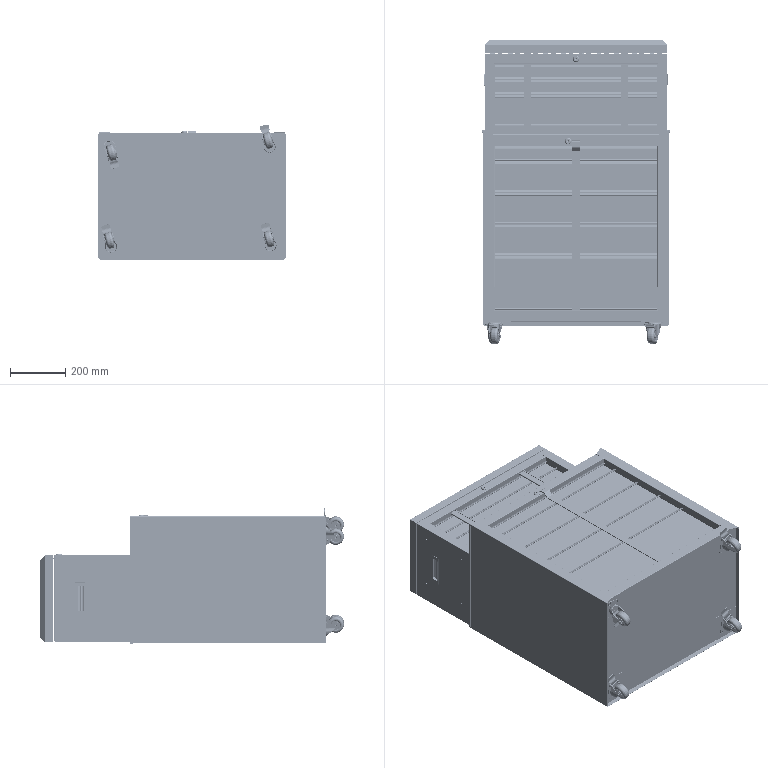Assembly | SolidWorks | mm | 91 component files | 95 solids | 8380 faces | box 675.6 x 1097.13 x 487.94 mm | volume 6787834 mm3 | plane 4464 | cylinder 3108 | spline 614 | torus 142 | cone 52 | commonest cylinder face diameters 4 x508 1 x387 2 x248 8 x224 3 x199 4.7 x186 5 x164 2.4 x130
Bill of materials:
Chapa Guantera Duesco | 2 | Plain Carbon Steel | Short cylindrical body with a wider flanged head with a chamfered edge. The shank has helical thread-like grooves interrupted by two flats on opposite sides. The end face has a slotted keyway-style recess, and a small rectangular tab sticks out of the opposite end.
Corredera A 400 | 10 | Plain Carbon Steel | Long, narrow formed channel (C-profile) with rounded bends and short return lips. The web has a row of pierced features: rectangular hook-like cut-outs, each with small round holes and slots around it, set in two groups near each end. There are notches at the ends.
Lengueta Chapa Guantera Duesco B | 1 | Plain Carbon Steel | Flat obround (stadium-shaped) plate with an eight-point star-shaped through cut-out near one end. A small cylindrical pin sits at the centre of the cut-out and sticks out a little below the plate.
Corredera C 400 | 10 | Plain Carbon Steel | Long, slender formed channel with rounded bends and short return flanges. It has three evenly spaced groups of small perforations along the web and a notch at one end.
PM-CAJ-P51 | 3 | Plain Carbon Steel | Long, narrow formed sheet profile. A flat base runs into an angled step and an upright leg at one edge. At the other edge it bends up into a side wall that ends in a folded-back (hemmed) angled lip. There are no visible holes.
PM-CAJ-P56 | 1 | Plain Carbon Steel | Rectangular sheet panel with a narrow perpendicular flange along one short edge. The flange has three small round holes in a line. There is also a small folded return along the top edge at one corner.
PM-CAJ-P54 | 4 | Plain Carbon Steel | Long formed sheet profile with a wide flat base. One edge has an angled step and an upright leg. The other edge has a vertical wall ending in a hemmed angled lip. There are no visible holes.
PM-CAJ-P57 | 3 | Plain Carbon Steel | Rectangular sheet panel with right-angle flanges along both short edges, forming a shallow U or tray shape seen from above. Each flange has three small round holes in a line.
PM-CAJ-P58 | 1 | Plain Carbon Steel | Rectangular sheet panel with deep right-angle flanges along both short edges, forming a U-shaped shell. Each flange has three small round holes in a line.
PM-CAJ-P59 | 1 | Plain Carbon Steel | Wide, long formed sheet profile. A large flat base has an angled step and an upright leg at one edge, and a vertical wall with a hemmed angled lip at the other edge. There are no visible holes.
PM-CAJ-P33 | 1 | Plain Carbon Steel | Rectangular sheet panel. Shallow flanges are folded along the bottom edge and both side edges, and the top edge has a folded channel-like return (a U-shaped hook). There are no visible holes.
PM-CAJ-P34 | 1 | Plain Carbon Steel | U-shaped formed sheet tray: a flat rectangular base with two tall parallel side walls. Each wall has a small inward lip along its top edge. Both walls have a few very small holes.
PM-CAJ-P35 | 1 | Plain Carbon Steel | Thin rectangular sheet panel with its top edge bent into an overhanging hooked lip; the lip's top face has one small rounded hole and a short slot next to it.
PM-CAJ-P60 | 4 | Plain Carbon Steel | Plain flat, roughly square thin plate.
PM-CAJ-P61 | 1 | Plain Carbon Steel | Long, narrow flat strip. One end has a raised step (joggle) and ends in a bent-down tab with a small window. The plan view shows a rectangular notch on one side and rounded corners at one end.
PM-CAJ-P62_MIR | 1 | Plain Carbon Steel | Sheet-metal channel-section panel: a large flat web with flanges along the top and bottom long edges, each ending in a short return lip. The web has a grid of small holes, and each flange has holes near its ends.
PM-CAJ-P62 | 1 | Plain Carbon Steel | Sheet-metal channel-section panel with top and bottom flanges ending in outward lips, a grid of small holes in the web, and holes in the flanges.
Pieza1 | 4 | Plain Carbon Steel | Wheel-like solid of revolution with a rounded, crowned outer tread, a recessed face with stepped concentric hub bosses, and a central through bore.
Pieza2 | 4 | Plain Carbon Steel | Rectangular plate with rounded corners and four obround slots near the corners. In the center, a shallow circular domed boss sticks out from one face, with a matching circular recess seen from the other face.
Pieza3 | 4 | Plain Carbon Steel | Bracket with two parallel side plates joined by a curved, scoop-like base. Each side plate has a lower through hole, and two cylindrical cross rods span the plates near the top.
Pieza4 | 4 | Plain Carbon Steel | Formed sheet bracket: a curved, S-profiled plate with rounded corners and two bent-down legs near one end, each leg with a round hole.
Bisagra de Piano 650mm | 2 | Plain Carbon Steel | Long thin flat strip with a row of ten small, evenly spaced raised tabs along its length. One long edge is rolled into an almost closed circular curl.
Corredera A 250 | 6 | Plain Carbon Steel | Elongated lipped C-channel upright. Its web has a repeating pattern of three U-shaped cutouts, each around a round hole and a short slot, with small holes between them. Small slots are at the top end, and three side-by-side cylinders sit inside the channel near the bottom end.
Lengueta Chapa Guantera Duesco A | 1 | Plain Carbon Steel | Flat, obround (stadium-shaped) lever-like plate with a joggled offset in the middle. One end has an eight-pointed star-shaped through hole with a small central pin; the other end has an angled open slot from the edge.
MANIJA  DE INCRUSTAR 115X40mm ACERO | 2 | Plain Carbon Steel | Rectangular plate with rounded corners and a raised rim, with a deep rectangular pocket behind it. The pocket's back face has vertical flutes, and a flat ledge with a small hole sits at one end.
Corredera C 250 | 6 | Plain Carbon Steel | Long, narrow formed strip. The end view shows a lipped channel (C-section) profile. The web has a pattern of small round holes and short slots near each end, and one end has a rectangular notch.
PM-CAJ-P36 | 2 | Plain Carbon Steel | Flat rectangular sheet panel with short bent flanges at both ends. One end flange has two small round holes.
PM-CAJ-P53 | 1 | Plain Carbon Steel | Rectangular sheet panel with wider bent flanges at both ends, giving a shallow U shape in plan. Each flange has two small holes.
PM-CAJ-P37 | 1 | Plain Carbon Steel | U-shaped sheet tray: a flat base with two upright end walls. Each wall has a central rectangular cutout, four small corner holes, and a short flange turned outward at the top edge.
PM-CAJ-P38 | 1 | Plain Carbon Steel | Rectangular sheet panel with a hook-shaped (J/inverted-L) fold along the top edge and narrow side returns. The top fold has two rectangular slots and one round hole near the middle.
PM-CAJ-P39 | 1 | Plain Carbon Steel | Rectangular sheet panel with a hook-shaped fold along the top edge and narrow side returns. It has no visible holes or slots.
PM-CAJ-P50 | 1 | Plain Carbon Steel | Shallow rectangular tray or frame: a flat panel surrounded by perimeter walls, with beveled outer edges. A small slot sits at the middle of one long edge, and a ledge runs along the opposite long side.
PM-CAJ-P52 | 2 | Plain Carbon Steel | Hat-section sheet part: a rectangular web with two perpendicular side walls ending in outward-turned flanges. Each flange has two holes, and the web has six holes in a 2x3 pattern.
PM-CAJ-P55 | 2 | Plain Carbon Steel | Long, thin channel strip. The end view shows a wide, shallow C-section with rounded corners and short inturned lips; the ends appear cut slightly at an angle or chamfered.
Tuerca Chapa Guantera Duesco | 1 | Plain Carbon Steel | Thin hexagonal ring: a flat hexagonal outline with a large central round bore, giving narrow walls at the flats.
Mates: